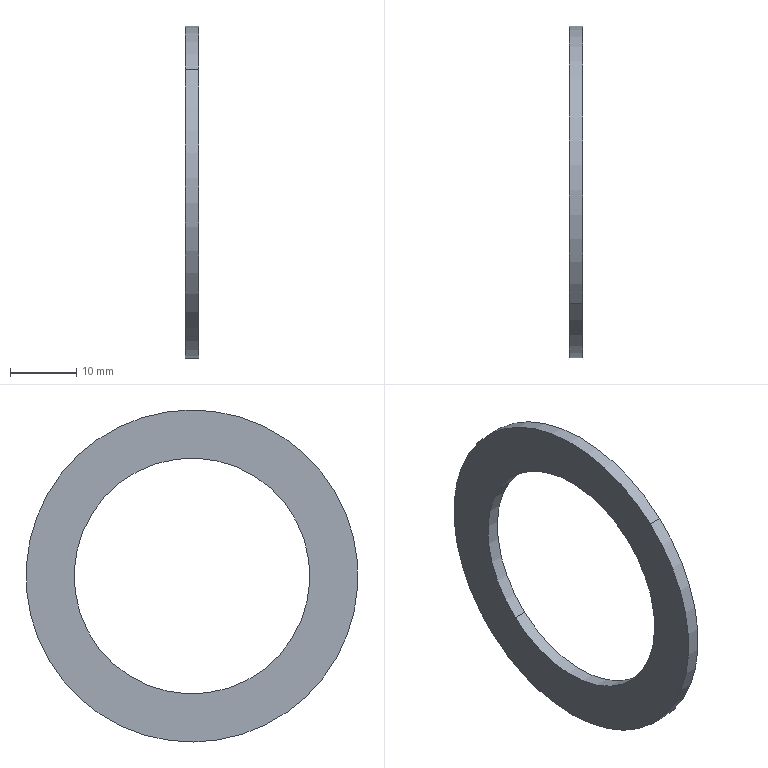Component | SolidWorks | 2-10-10WorkpieceAxisAssembly-1_2-10-6BearingShim-1 | 1 solid | 6 faces | box 2 x 50 x 50 mm | volume 1947 mm3 | cylinder 4 | plane 2 | commonest cylinder face diameters 35.5 x2 50 x2
build123d program:
from build123d import *

# Parameters (mm, degrees)
SKETCH1_R      = 25
SKETCH1_R_2    = 17.75
EXTRUDE1_DEPTH = 2


with BuildPart() as part:
    # Sketch1 → Extrude1 (new body)
    with BuildSketch(Plane(origin=(0, 0, 0), x_dir=(1, 0, 0), z_dir=(0, 1, 0))):
        with Locations(Location((0, 0, 0), (0, 0, 270))):
            Circle(SKETCH1_R)
        with Locations(Location((0, 0, 0), (0, 0, 270))):
            Circle(SKETCH1_R_2, mode=Mode.SUBTRACT)
    extrude(amount=EXTRUDE1_DEPTH)


solid = part.part

# Placed as in the assembly
solid = solid.moved(Location((-203.809, -4.181, 0), (0, 0, 90)))
STEP:
#1=COLOUR_RGB('',0.7922,0.8196,0.9333);
#2=FILL_AREA_STYLE_COLOUR('',#1);
#3=FILL_AREA_STYLE('',(#2));
#4=SURFACE_STYLE_FILL_AREA(#3);
#5=SURFACE_SIDE_STYLE('',(#4));
#6=SURFACE_STYLE_USAGE(.BOTH.,#5);
#7=PRESENTATION_STYLE_ASSIGNMENT((#6));
#8=CARTESIAN_POINT('',(-8.103,-0.6341,0.5176));
#9=VERTEX_POINT('',#8);
#10=CARTESIAN_POINT('',(-8.103,0.3049,-0.5176));
#11=VERTEX_POINT('',#10);
#12=CARTESIAN_POINT('',(-8.103,-0.1646,-0.));
#13=DIRECTION('',(-1.,0.,-0.));
#14=DIRECTION('',(0.,0.6719,-0.7407));
#15=AXIS2_PLACEMENT_3D('',#12,#13,#14);
#16=CIRCLE('',#15,0.6988);
#17=EDGE_CURVE('',#9,#11,#16,.T.);
#18=ORIENTED_EDGE('',*,*,#17,.T.);
#19=CARTESIAN_POINT('',(-8.024,0.3049,-0.5176));
#20=VERTEX_POINT('',#19);
#21=CARTESIAN_POINT('',(-8.103,0.3049,-0.5176));
#22=DIRECTION('',(1.,-0.,0.));
#23=VECTOR('',#22,39.37);
#24=LINE('',#21,#23);
#25=EDGE_CURVE('',#11,#20,#24,.T.);
#26=ORIENTED_EDGE('',*,*,#25,.T.);
#27=CARTESIAN_POINT('',(-8.024,-0.6341,0.5176));
#28=VERTEX_POINT('',#27);
#29=CARTESIAN_POINT('',(-8.024,-0.1646,-0.));
#30=DIRECTION('',(-1.,0.,-0.));
#31=DIRECTION('',(0.,0.6719,-0.7407));
#32=AXIS2_PLACEMENT_3D('',#29,#30,#31);
#33=CIRCLE('',#32,0.6988);
#34=EDGE_CURVE('',#28,#20,#33,.T.);
#35=ORIENTED_EDGE('',*,*,#34,.F.);
#36=CARTESIAN_POINT('',(-8.103,-0.6341,0.5176));
#37=DIRECTION('',(1.,-0.,0.));
#38=VECTOR('',#37,39.37);
#39=LINE('',#36,#38);
#40=EDGE_CURVE('',#9,#28,#39,.T.);
#41=ORIENTED_EDGE('',*,*,#40,.F.);
#42=EDGE_LOOP('',(#18,#26,#35,#41));
#43=FACE_OUTER_BOUND('',#42,.T.);
#44=CARTESIAN_POINT('',(-8.103,-0.1646,-0.));
#45=DIRECTION('',(1.,-0.,0.));
#46=DIRECTION('',(0.,-0.6719,0.7407));
#47=AXIS2_PLACEMENT_3D('',#44,#45,#46);
#48=CYLINDRICAL_SURFACE('',#47,0.6988);
#49=ADVANCED_FACE('',(#43),#48,.F.);
#50=CARTESIAN_POINT('',(-8.103,0.4967,-0.729));
#51=VERTEX_POINT('',#50);
#52=CARTESIAN_POINT('',(-8.103,-0.8259,0.729));
#53=VERTEX_POINT('',#52);
#54=CARTESIAN_POINT('',(-8.103,-0.1646,-0.));
#55=DIRECTION('',(-1.,0.,-0.));
#56=DIRECTION('',(0.,0.6719,-0.7407));
#57=AXIS2_PLACEMENT_3D('',#54,#55,#56);
#58=CIRCLE('',#57,0.9843);
#59=EDGE_CURVE('',#51,#53,#58,.T.);
#60=ORIENTED_EDGE('',*,*,#59,.F.);
#61=CARTESIAN_POINT('',(-8.024,0.4967,-0.729));
#62=VERTEX_POINT('',#61);
#63=CARTESIAN_POINT('',(-8.103,0.4967,-0.729));
#64=DIRECTION('',(1.,-0.,0.));
#65=VECTOR('',#64,39.37);
#66=LINE('',#63,#65);
#67=EDGE_CURVE('',#51,#62,#66,.T.);
#68=ORIENTED_EDGE('',*,*,#67,.T.);
#69=CARTESIAN_POINT('',(-8.024,-0.8259,0.729));
#70=VERTEX_POINT('',#69);
#71=CARTESIAN_POINT('',(-8.024,-0.1646,-0.));
#72=DIRECTION('',(-1.,0.,-0.));
#73=DIRECTION('',(0.,0.6719,-0.7407));
#74=AXIS2_PLACEMENT_3D('',#71,#72,#73);
#75=CIRCLE('',#74,0.9843);
#76=EDGE_CURVE('',#62,#70,#75,.T.);
#77=ORIENTED_EDGE('',*,*,#76,.T.);
#78=CARTESIAN_POINT('',(-8.103,-0.8259,0.729));
#79=DIRECTION('',(1.,-0.,0.));
#80=VECTOR('',#79,39.37);
#81=LINE('',#78,#80);
#82=EDGE_CURVE('',#53,#70,#81,.T.);
#83=ORIENTED_EDGE('',*,*,#82,.F.);
#84=EDGE_LOOP('',(#60,#68,#77,#83));
#85=FACE_OUTER_BOUND('',#84,.T.);
#86=CARTESIAN_POINT('',(-8.103,-0.1646,-0.));
#87=DIRECTION('',(1.,-0.,0.));
#88=DIRECTION('',(0.,-0.6719,0.7407));
#89=AXIS2_PLACEMENT_3D('',#86,#87,#88);
#90=CYLINDRICAL_SURFACE('',#89,0.9843);
#91=ADVANCED_FACE('',(#85),#90,.T.);
#92=CARTESIAN_POINT('',(-8.103,-0.1646,-0.));
#93=DIRECTION('',(-1.,0.,-0.));
#94=DIRECTION('',(0.,0.6719,-0.7407));
#95=AXIS2_PLACEMENT_3D('',#92,#93,#94);
#96=CIRCLE('',#95,0.9843);
#97=EDGE_CURVE('',#53,#51,#96,.T.);
#98=ORIENTED_EDGE('',*,*,#97,.T.);
#99=ORIENTED_EDGE('',*,*,#59,.T.);
#100=EDGE_LOOP('',(#98,#99));
#101=FACE_OUTER_BOUND('',#100,.T.);
#102=ORIENTED_EDGE('',*,*,#17,.F.);
#103=CARTESIAN_POINT('',(-8.103,-0.1646,-0.));
#104=DIRECTION('',(-1.,0.,-0.));
#105=DIRECTION('',(0.,0.6719,-0.7407));
#106=AXIS2_PLACEMENT_3D('',#103,#104,#105);
#107=CIRCLE('',#106,0.6988);
#108=EDGE_CURVE('',#11,#9,#107,.T.);
#109=ORIENTED_EDGE('',*,*,#108,.F.);
#110=EDGE_LOOP('',(#102,#109));
#111=FACE_BOUND('',#110,.T.);
#112=CARTESIAN_POINT('',(-8.103,-0.1646,-0.));
#113=DIRECTION('',(-1.,0.,-0.));
#114=DIRECTION('',(0.,0.6719,-0.7407));
#115=AXIS2_PLACEMENT_3D('',#112,#113,#114);
#116=PLANE('',#115);
#117=ADVANCED_FACE('',(#101,#111),#116,.T.);
#118=CARTESIAN_POINT('',(-8.024,-0.1646,-0.));
#119=DIRECTION('',(-1.,0.,-0.));
#120=DIRECTION('',(0.,0.6719,-0.7407));
#121=AXIS2_PLACEMENT_3D('',#118,#119,#120);
#122=CIRCLE('',#121,0.9843);
#123=EDGE_CURVE('',#70,#62,#122,.T.);
#124=ORIENTED_EDGE('',*,*,#123,.F.);
#125=ORIENTED_EDGE('',*,*,#76,.F.);
#126=EDGE_LOOP('',(#124,#125));
#127=FACE_OUTER_BOUND('',#126,.T.);
#128=ORIENTED_EDGE('',*,*,#34,.T.);
#129=CARTESIAN_POINT('',(-8.024,-0.1646,-0.));
#130=DIRECTION('',(-1.,0.,-0.));
#131=DIRECTION('',(0.,0.6719,-0.7407));
#132=AXIS2_PLACEMENT_3D('',#129,#130,#131);
#133=CIRCLE('',#132,0.6988);
#134=EDGE_CURVE('',#20,#28,#133,.T.);
#135=ORIENTED_EDGE('',*,*,#134,.T.);
#136=EDGE_LOOP('',(#128,#135));
#137=FACE_BOUND('',#136,.T.);
#138=CARTESIAN_POINT('',(-8.024,-0.1646,-0.));
#139=DIRECTION('',(-1.,0.,-0.));
#140=DIRECTION('',(0.,0.6719,-0.7407));
#141=AXIS2_PLACEMENT_3D('',#138,#139,#140);
#142=PLANE('',#141);
#143=ADVANCED_FACE('',(#127,#137),#142,.F.);
#144=ORIENTED_EDGE('',*,*,#67,.F.);
#145=ORIENTED_EDGE('',*,*,#97,.F.);
#146=ORIENTED_EDGE('',*,*,#82,.T.);
#147=ORIENTED_EDGE('',*,*,#123,.T.);
#148=EDGE_LOOP('',(#144,#145,#146,#147));
#149=FACE_OUTER_BOUND('',#148,.T.);
#150=CARTESIAN_POINT('',(-8.103,-0.1646,-0.));
#151=DIRECTION('',(1.,-0.,0.));
#152=DIRECTION('',(0.,-0.6719,0.7407));
#153=AXIS2_PLACEMENT_3D('',#150,#151,#152);
#154=CYLINDRICAL_SURFACE('',#153,0.9843);
#155=ADVANCED_FACE('',(#149),#154,.T.);
#156=ORIENTED_EDGE('',*,*,#25,.F.);
#157=ORIENTED_EDGE('',*,*,#108,.T.);
#158=ORIENTED_EDGE('',*,*,#40,.T.);
#159=ORIENTED_EDGE('',*,*,#134,.F.);
#160=EDGE_LOOP('',(#156,#157,#158,#159));
#161=FACE_OUTER_BOUND('',#160,.T.);
#162=CARTESIAN_POINT('',(-8.103,-0.1646,-0.));
#163=DIRECTION('',(1.,-0.,0.));
#164=DIRECTION('',(0.,-0.6719,0.7407));
#165=AXIS2_PLACEMENT_3D('',#162,#163,#164);
#166=CYLINDRICAL_SURFACE('',#165,0.6988);
#167=ADVANCED_FACE('',(#161),#166,.F.);
#168=CLOSED_SHELL('',(#49,#91,#117,#143,#155,#167));
#169=MANIFOLD_SOLID_BREP('',#168);
#170=STYLED_ITEM('',(#7),#169);
#171=PRESENTATION_LAYER_ASSIGNMENT('','',(#170));
#172=(LENGTH_UNIT()NAMED_UNIT(*)SI_UNIT($,.METRE.));
#173=LENGTH_MEASURE_WITH_UNIT(LENGTH_MEASURE(0.0254),#172);
#174=DIMENSIONAL_EXPONENTS(1.,0.,0.,0.,0.,0.,0.);
#175=(CONVERSION_BASED_UNIT('',#173)LENGTH_UNIT()NAMED_UNIT(#174));
#176=UNCERTAINTY_MEASURE_WITH_UNIT(LENGTH_MEASURE(0.00001),#175,'','');
#177=(NAMED_UNIT(*)PLANE_ANGLE_UNIT()SI_UNIT($,.RADIAN.));
#178=(NAMED_UNIT(*)SI_UNIT($,.STERADIAN.)SOLID_ANGLE_UNIT());
#179=(GEOMETRIC_REPRESENTATION_CONTEXT(3)GLOBAL_UNCERTAINTY_ASSIGNED_CONTEXT((#176))GLOBAL_UNIT_ASSIGNED_CONTEXT((#175,#177,#178))REPRESENTATION_CONTEXT('',''));
#180=MECHANICAL_DESIGN_GEOMETRIC_PRESENTATION_REPRESENTATION('',(#170),#179);
#181=CARTESIAN_POINT('',(0.,0.,0.));
#182=DIRECTION('',(0.,0.,1.));
#183=DIRECTION('',(1.,0.,0.));
#184=AXIS2_PLACEMENT_3D('',#181,#182,#183);
#185=(LENGTH_UNIT()NAMED_UNIT(*)SI_UNIT($,.METRE.));
#186=LENGTH_MEASURE_WITH_UNIT(LENGTH_MEASURE(0.0254),#185);
#187=DIMENSIONAL_EXPONENTS(1.,0.,0.,0.,0.,0.,0.);
#188=(CONVERSION_BASED_UNIT('',#186)LENGTH_UNIT()NAMED_UNIT(#187));
#189=UNCERTAINTY_MEASURE_WITH_UNIT(LENGTH_MEASURE(0.00001),#188,'','');
#190=(NAMED_UNIT(*)PLANE_ANGLE_UNIT()SI_UNIT($,.RADIAN.));
#191=(NAMED_UNIT(*)SI_UNIT($,.STERADIAN.)SOLID_ANGLE_UNIT());
#192=(GEOMETRIC_REPRESENTATION_CONTEXT(3)GLOBAL_UNCERTAINTY_ASSIGNED_CONTEXT((#189))GLOBAL_UNIT_ASSIGNED_CONTEXT((#188,#190,#191))REPRESENTATION_CONTEXT('',''));
#193=ADVANCED_BREP_SHAPE_REPRESENTATION('',(#169,#184),#192);